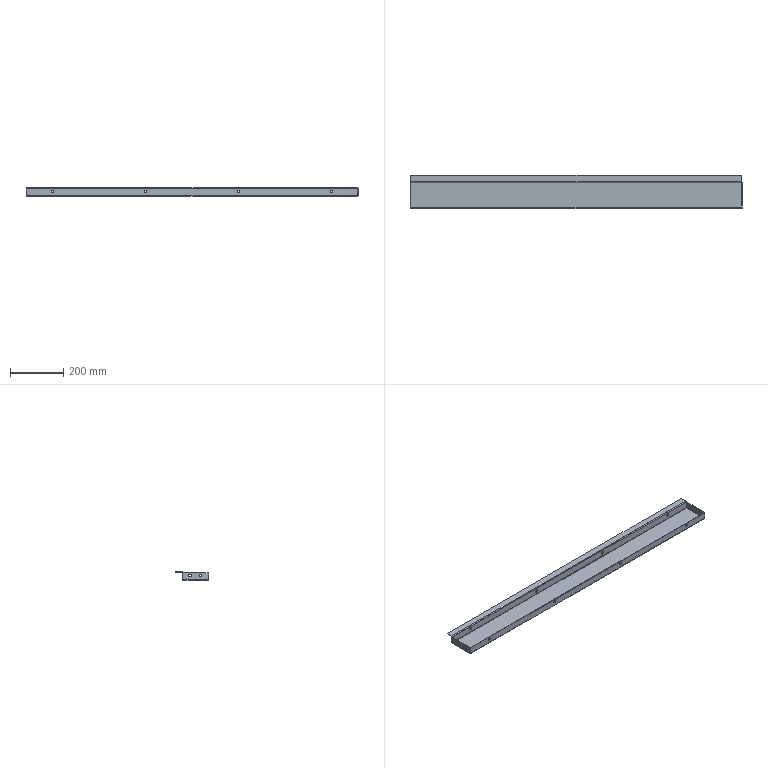Component | SolidWorks | 26BaseRearSidePlateI-1 | 1 solid | 70 faces | volume 453065 mm3 | cylinder 34 | plane 28 | spline 8 | commonest cylinder face diameters 10 x24 2 x5 6 x5